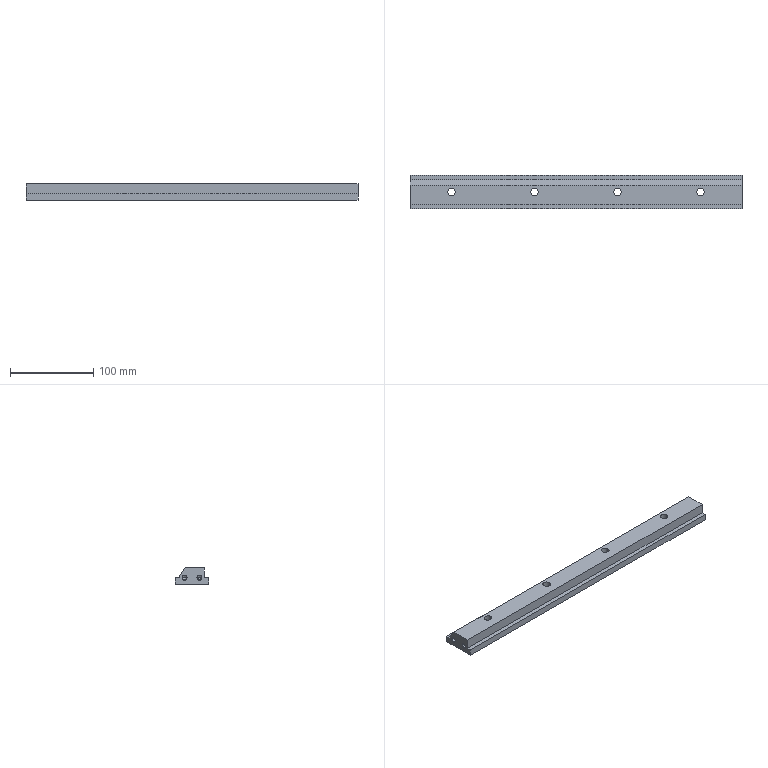Component | SolidWorks | 31FixedGuideRail-1 | 1 solid | 43 faces | box 400 x 40 x 20 mm | volume 248245 mm3 | cylinder 20 | plane 15 | cone 8 | commonest cylinder face diameters 14 x8 9 x8 5 x4
build123d program:
from build123d import *

# Parameters (mm, degrees)
SKETCH1_W                   = 40
SKETCH1_H                   = 20
BOSS_EXTRUDE1_DEPTH         = 400
SKETCH2_W                   = 5
SKETCH2_H                   = 12
CUT_EXTRUDE1_DEPTH          = 400
SKETCH3_R                   = 4.5
CUT_EXTRUDE2_DEPTH          = 60
SKETCH4_R                   = 7
CUT_EXTRUDE3_DEPTH          = 11
M6_TAPPED_HOLE1_D           = 5
M6_TAPPED_HOLE1_DEPTH       = 17
M6_TAPPED_HOLE1_CSINK_D     = 6.05
M6_TAPPED_HOLE1_CSINK_ANGLE = 90
M6_TAPPED_HOLE1_TIP         = 1.502


with BuildPart() as part:
    # Sketch1 → Boss-Extrude1 (new body)
    with BuildSketch(Plane.XY):
        Rectangle(SKETCH1_W, SKETCH1_H)
    extrude(amount=BOSS_EXTRUDE1_DEPTH)

    # Sketch2 → Cut-Extrude1 (cut)
    with BuildSketch(Plane.XY.offset(400)):
        Polygon((-20, 10), (-15, 10), (-15, 22), (-25, 22), (-25, -2), (-20, -2), align=None)
        Polygon((-15, 0), (-8, 10), (-15, 10), align=None)
        Polygon((25, 22), (15, 22), (15, 10), (20, 10), (20, -2), (25, -2), align=None)
        with Locations((17.5, 4)):
            Rectangle(SKETCH2_W, SKETCH2_H)
        Polygon((-15, -2), (-15, 0), (-15, 10), (-20, 10), (-20, -2), align=None)
    extrude(amount=-CUT_EXTRUDE1_DEPTH, mode=Mode.SUBTRACT)

    # Sketch3 → Cut-Extrude2 (cut)
    with BuildSketch(Plane(origin=(0, 10, 0), x_dir=(1, 0, 0), z_dir=(0, 1, 0))):
        with Locations(Location((0, -350, 0), (0, 0, 270))):
            Circle(SKETCH3_R)
        with Locations(Location((0, -250, 0), (0, 0, 270))):
            Circle(SKETCH3_R)
        with Locations(Location((0, -150, 0), (0, 0, 270))):
            Circle(SKETCH3_R)
        with Locations(Location((0, -50, 0), (0, 0, 270))):
            Circle(SKETCH3_R)
    extrude(amount=-CUT_EXTRUDE2_DEPTH, mode=Mode.SUBTRACT)

    # Sketch4 → Cut-Extrude3 (cut)
    with BuildSketch(Plane.XZ.offset(10)):
        with Locations(Location((0, 50, 0), (0, 0, 270))):
            Circle(SKETCH4_R)
        with Locations(Location((0, 150, 0), (0, 0, 270))):
            Circle(SKETCH4_R)
        with Locations(Location((0, 250, 0), (0, 0, 270))):
            Circle(SKETCH4_R)
        with Locations(Location((0, 350, 0), (0, 0, 270))):
            Circle(SKETCH4_R)
    extrude(amount=-CUT_EXTRUDE3_DEPTH, mode=Mode.SUBTRACT)

    # M6 Tapped Hole1
    with Locations(Plane.XY.offset(400)):
        with Locations((-9, -2), (9, -2)):
            CounterSinkHole(M6_TAPPED_HOLE1_D / 2, M6_TAPPED_HOLE1_CSINK_D / 2, depth=M6_TAPPED_HOLE1_DEPTH, counter_sink_angle=M6_TAPPED_HOLE1_CSINK_ANGLE)
            with Locations((0, 0, -(M6_TAPPED_HOLE1_DEPTH + M6_TAPPED_HOLE1_TIP / 2))):  # 118° drill point
                Cone(0, M6_TAPPED_HOLE1_D / 2, M6_TAPPED_HOLE1_TIP, mode=Mode.SUBTRACT)


solid = part.part

# Placed as in the assembly
solid = solid.moved(Location((200, 57, -90), (90, -90, 0)))